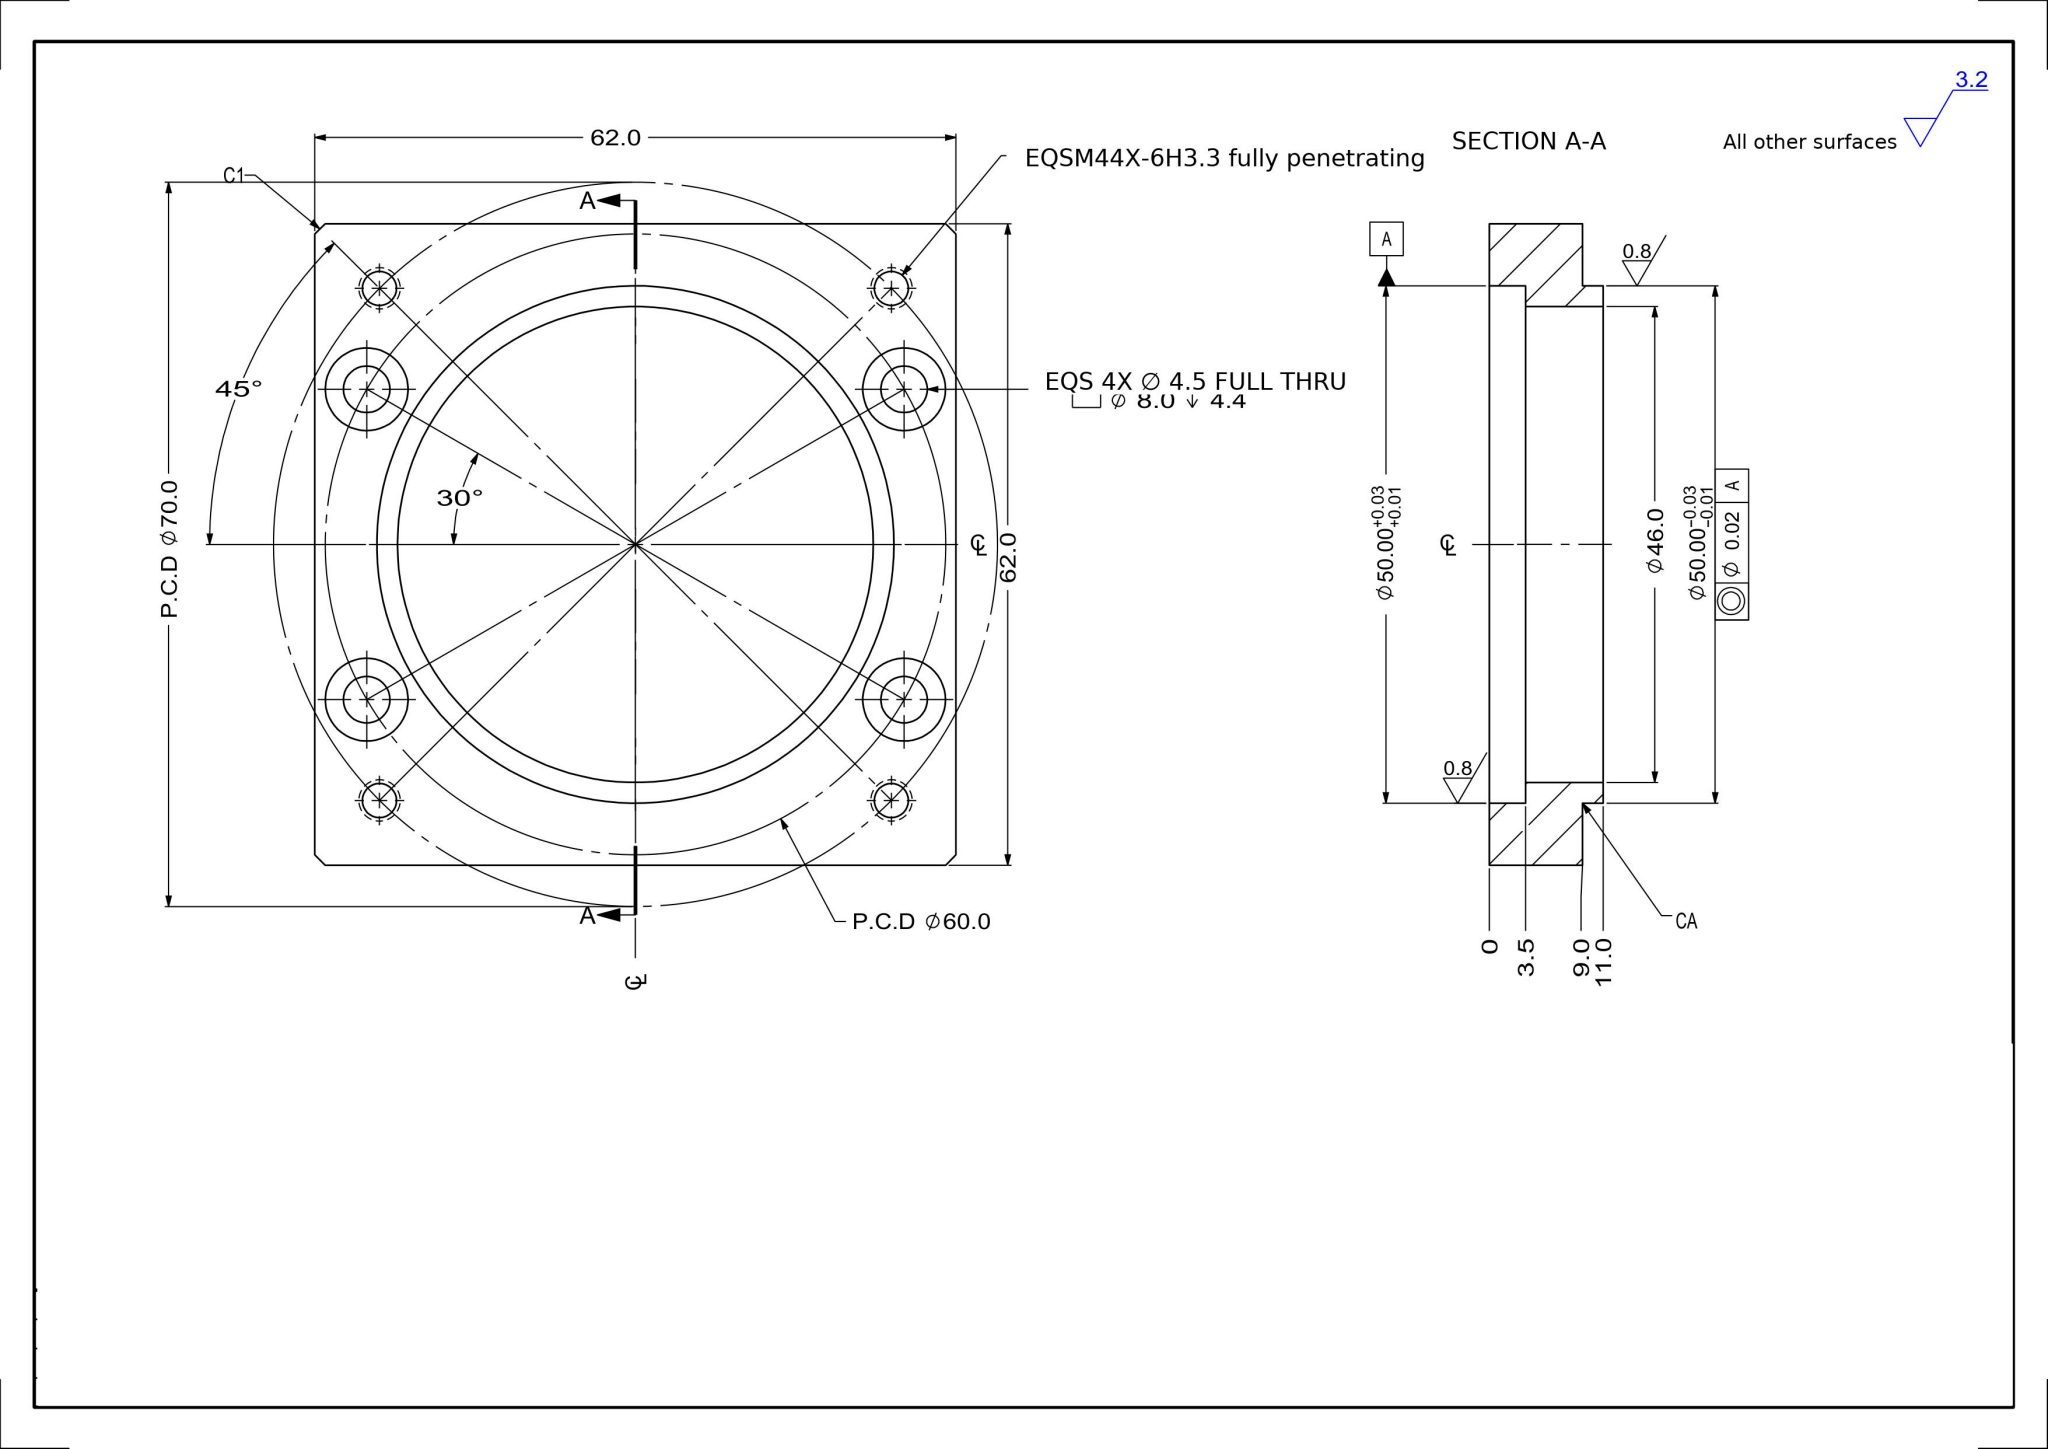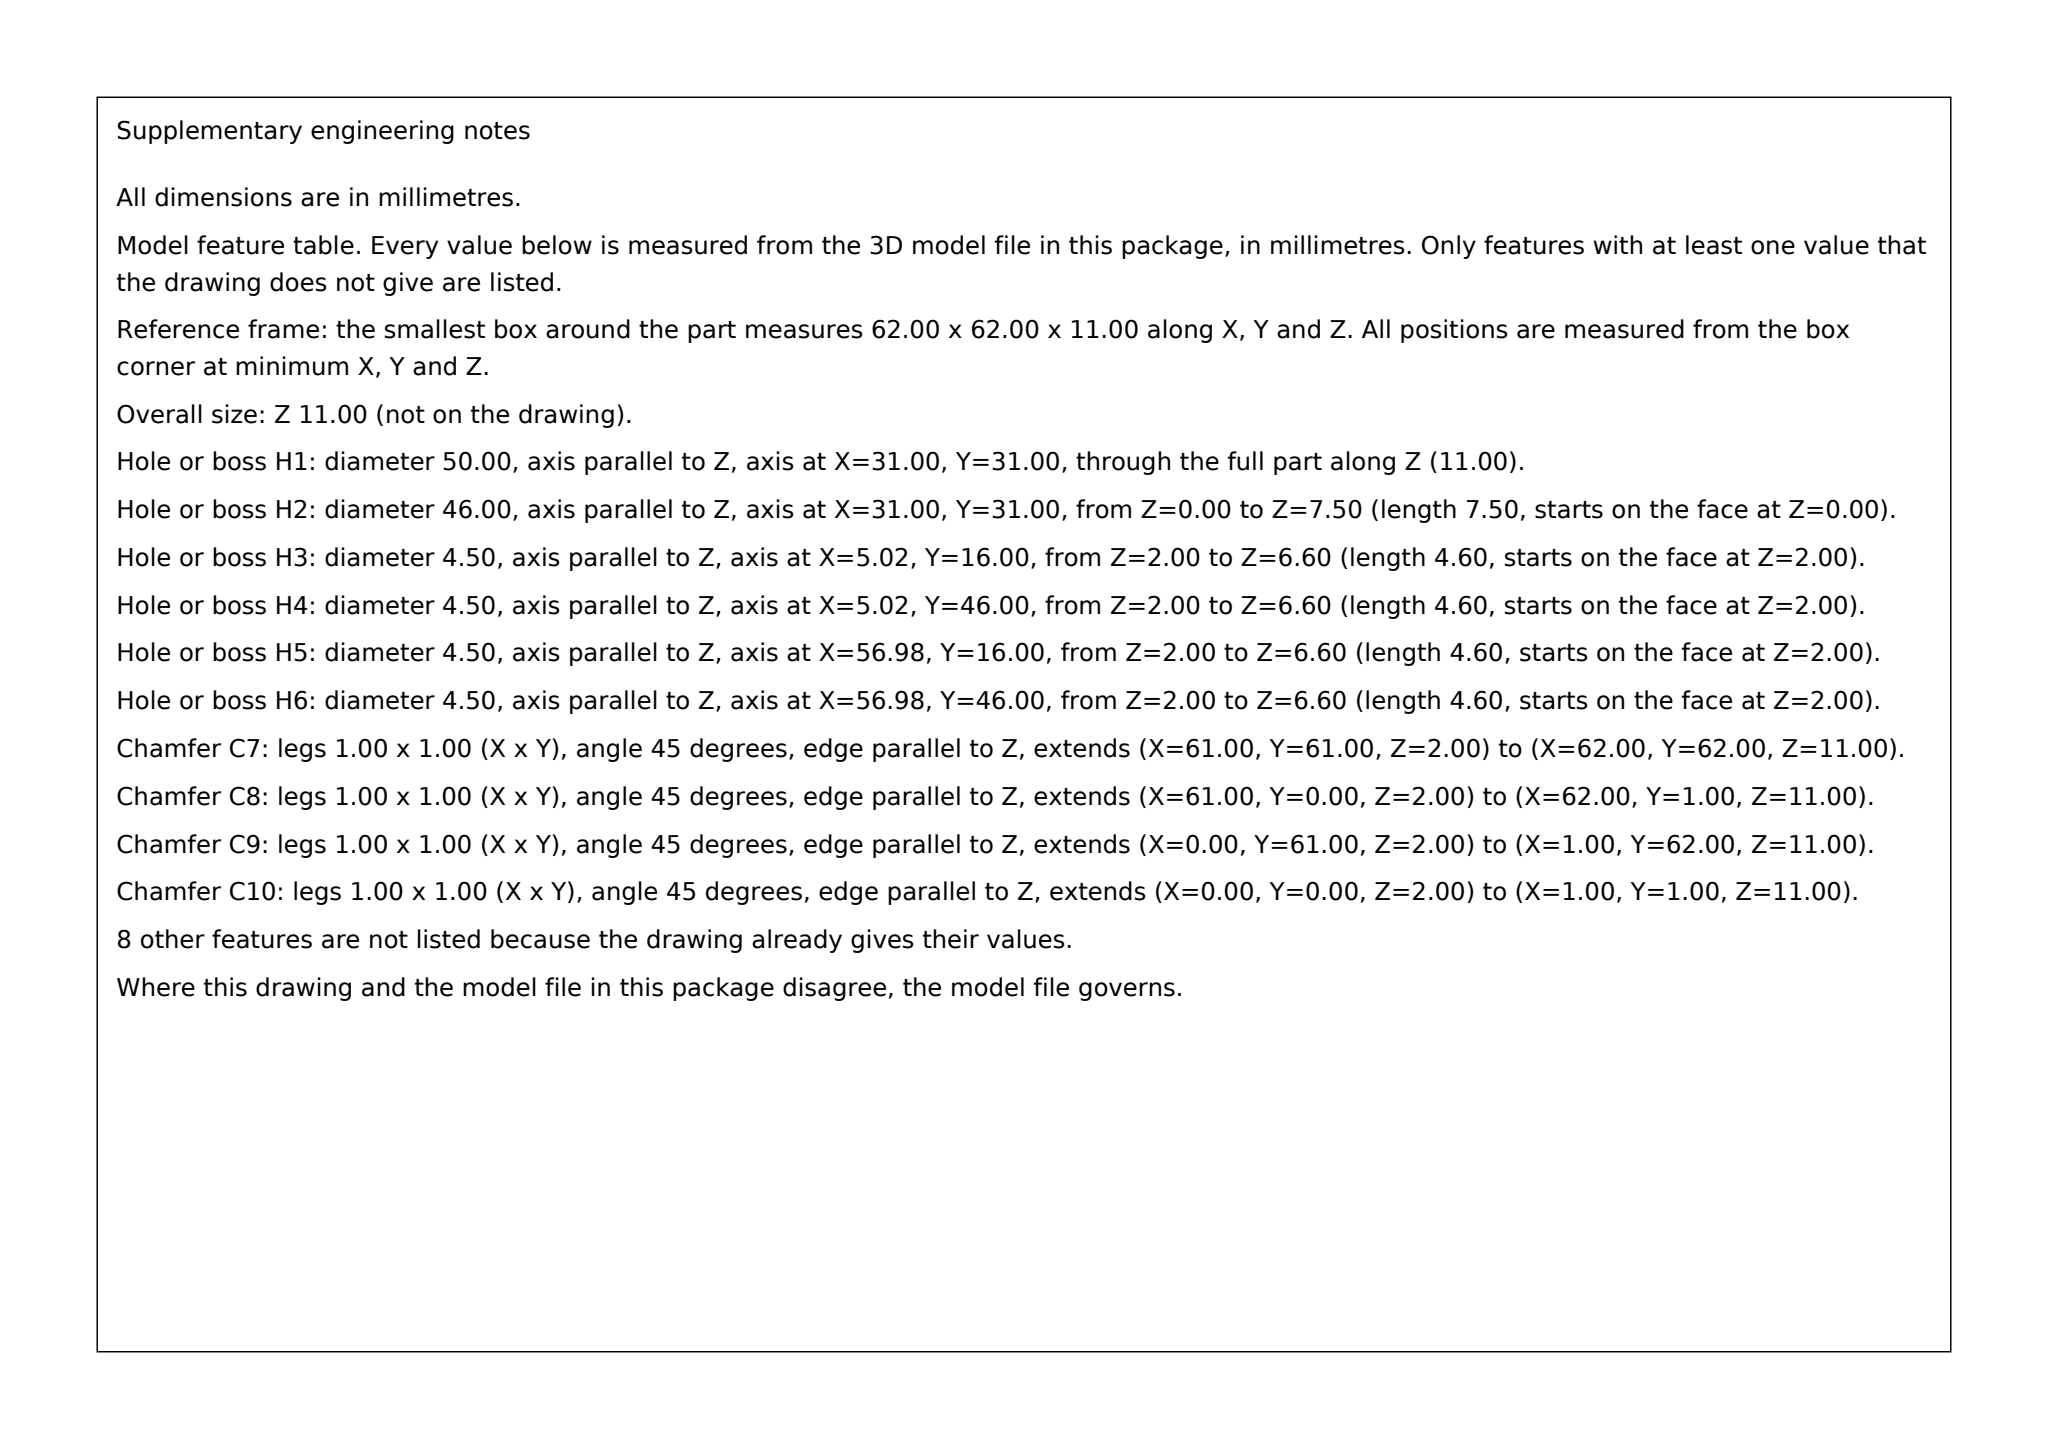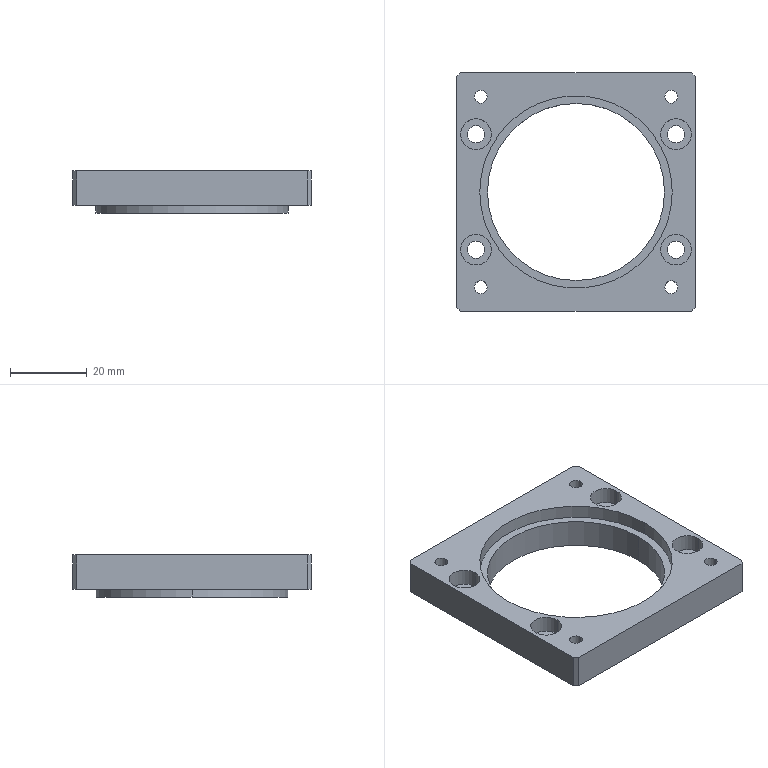Part | SolidWorks | mm | 1 solid | 46 faces | box 62 x 62 x 11 mm | volume 17683 mm3 | cylinder 30 | plane 16 | commonest cylinder face diameters 8 x8 4.5 x8 3.3 x8 50 x4 46 x2
build123d program:
from build123d import *

# Parameters (mm, degrees)
SKETCH1_W                                       = 62
SKETCH1_H                                       = 62
BOSS_EXTRUDE1_DEPTH                             = 5.5
SKETCH2_W                                       = 62
SKETCH2_H                                       = 62
SKETCH2_R                                       = 25
CUT_EXTRUDE1_DEPTH                              = 2
SKETCH3_R                                       = 23
CUT_EXTRUDE2_DEPTH                              = 46.2
CUT_EXTRUDE3_START                              = -3.5
SKETCH4_R                                       = 25
CUT_EXTRUDE3_DEPTH                              = 3.5
M4_TAPPED_HOLE1_D                               = 3.3
M4_HEX_SOCKET_HEAD_CAP_SCREW_CBORE1_D           = 4.5
M4_HEX_SOCKET_HEAD_CAP_SCREW_CBORE1_CBORE_D     = 8
M4_HEX_SOCKET_HEAD_CAP_SCREW_CBORE1_CBORE_DEPTH = 4.4
CHAMFER1_SIZE                                   = 1


with BuildPart() as part:
    # Sketch1 → Boss-Extrude1 (new, symmetric)
    with BuildSketch(Plane.XY):
        Rectangle(SKETCH1_W, SKETCH1_H)
    extrude(amount=BOSS_EXTRUDE1_DEPTH, both=True)

    # Sketch2 → Cut-Extrude1 (cut)
    with BuildSketch(Plane(origin=(0, 0, -5.5), x_dir=(-1, 0, 0), z_dir=(0, 0, -1))):
        Rectangle(SKETCH2_W, SKETCH2_H)
        Circle(SKETCH2_R, mode=Mode.SUBTRACT)
    extrude(amount=-CUT_EXTRUDE1_DEPTH, mode=Mode.SUBTRACT)

    # Sketch3 → Cut-Extrude2 (cut, through all)
    with BuildSketch(Plane(origin=(0, 0, -5.5), x_dir=(-1, 0, 0), z_dir=(0, 0, -1))):
        Circle(SKETCH3_R)
    extrude(amount=-CUT_EXTRUDE2_DEPTH, mode=Mode.SUBTRACT)

    # Sketch4 → Cut-Extrude3 (cut)
    with BuildSketch(Plane.XY.offset(5.5).offset(CUT_EXTRUDE3_START)):
        with Locations(Location((0, 0, 0), (0, 0, 180))):
            Circle(SKETCH4_R)
    extrude(amount=CUT_EXTRUDE3_DEPTH, mode=Mode.SUBTRACT)

    # M4 Tapped Hole1 (through all)
    with Locations(Plane.XY.offset(5.5)):
        with Locations((24.75, -24.747), (-24.75, -24.747), (24.75, 24.747), (-24.75, 24.747)):
            Hole(M4_TAPPED_HOLE1_D / 2)

    # M4 Hex Socket Head Cap Screw CBORE1 (through all)
    with Locations(Plane.XY.offset(5.5)):
        with Locations((25.98, -15), (25.98, 15), (-25.98, -15), (-25.98, 15)):
            CounterBoreHole(M4_HEX_SOCKET_HEAD_CAP_SCREW_CBORE1_D / 2, M4_HEX_SOCKET_HEAD_CAP_SCREW_CBORE1_CBORE_D / 2, M4_HEX_SOCKET_HEAD_CAP_SCREW_CBORE1_CBORE_DEPTH)

    # Chamfer1
    chamfer1_edges = [part.edges().sort_by_distance(p)[0] for p in [
        (31, -31, 1),
        (-31, -31, 1),
        (-31, 31, 1),
        (31, 31, 1),
    ]]
    chamfer(chamfer1_edges, length=CHAMFER1_SIZE)


solid = part.part